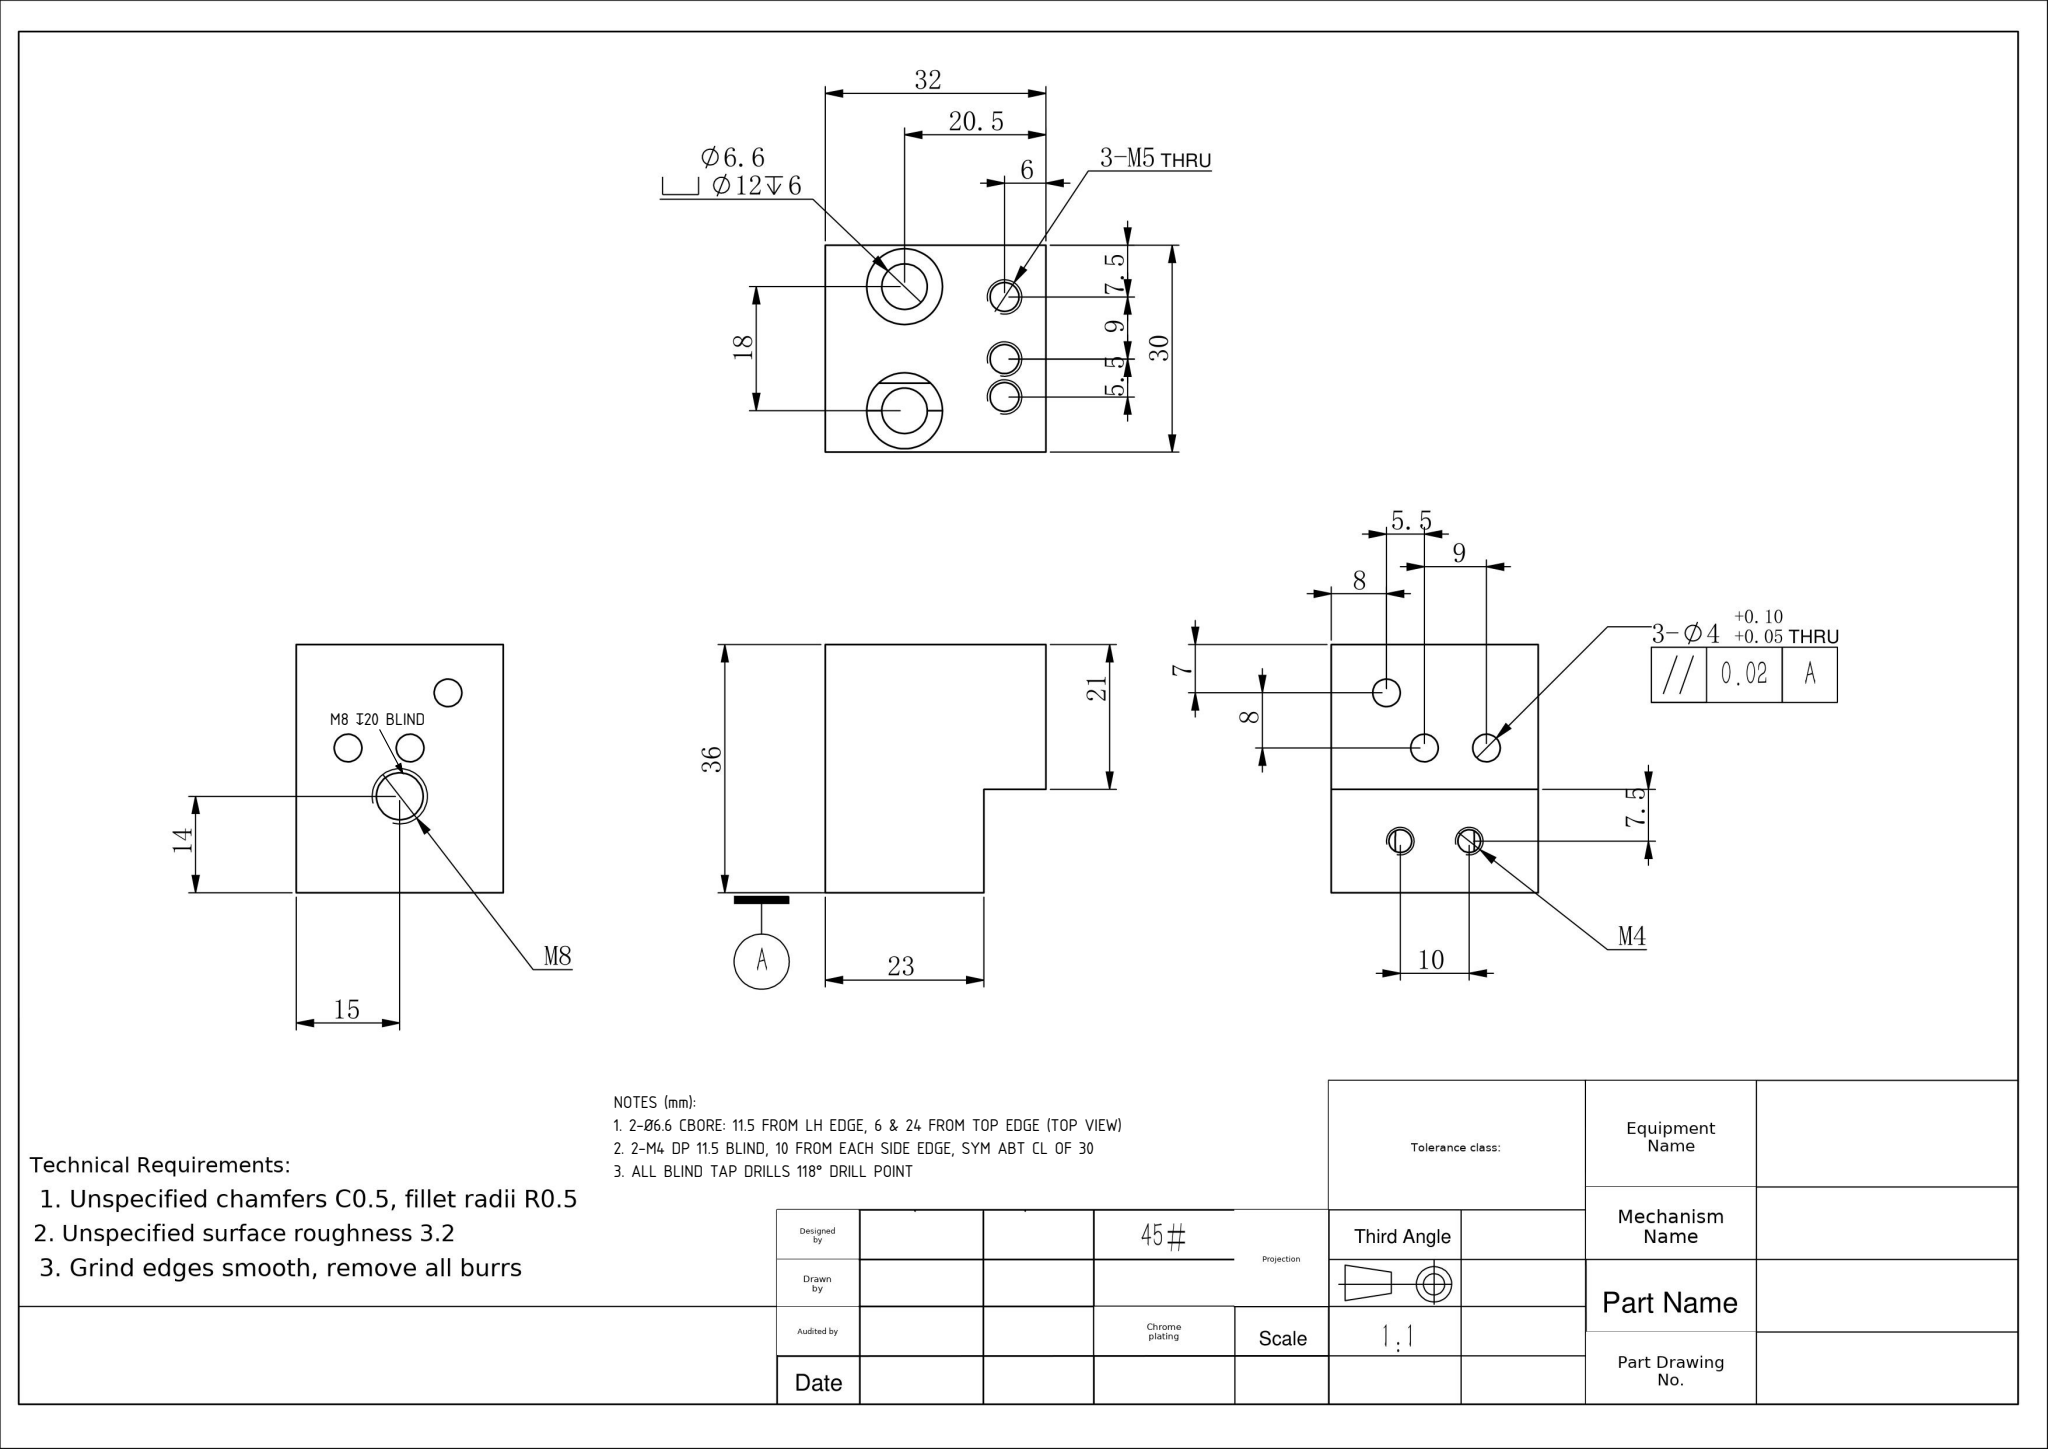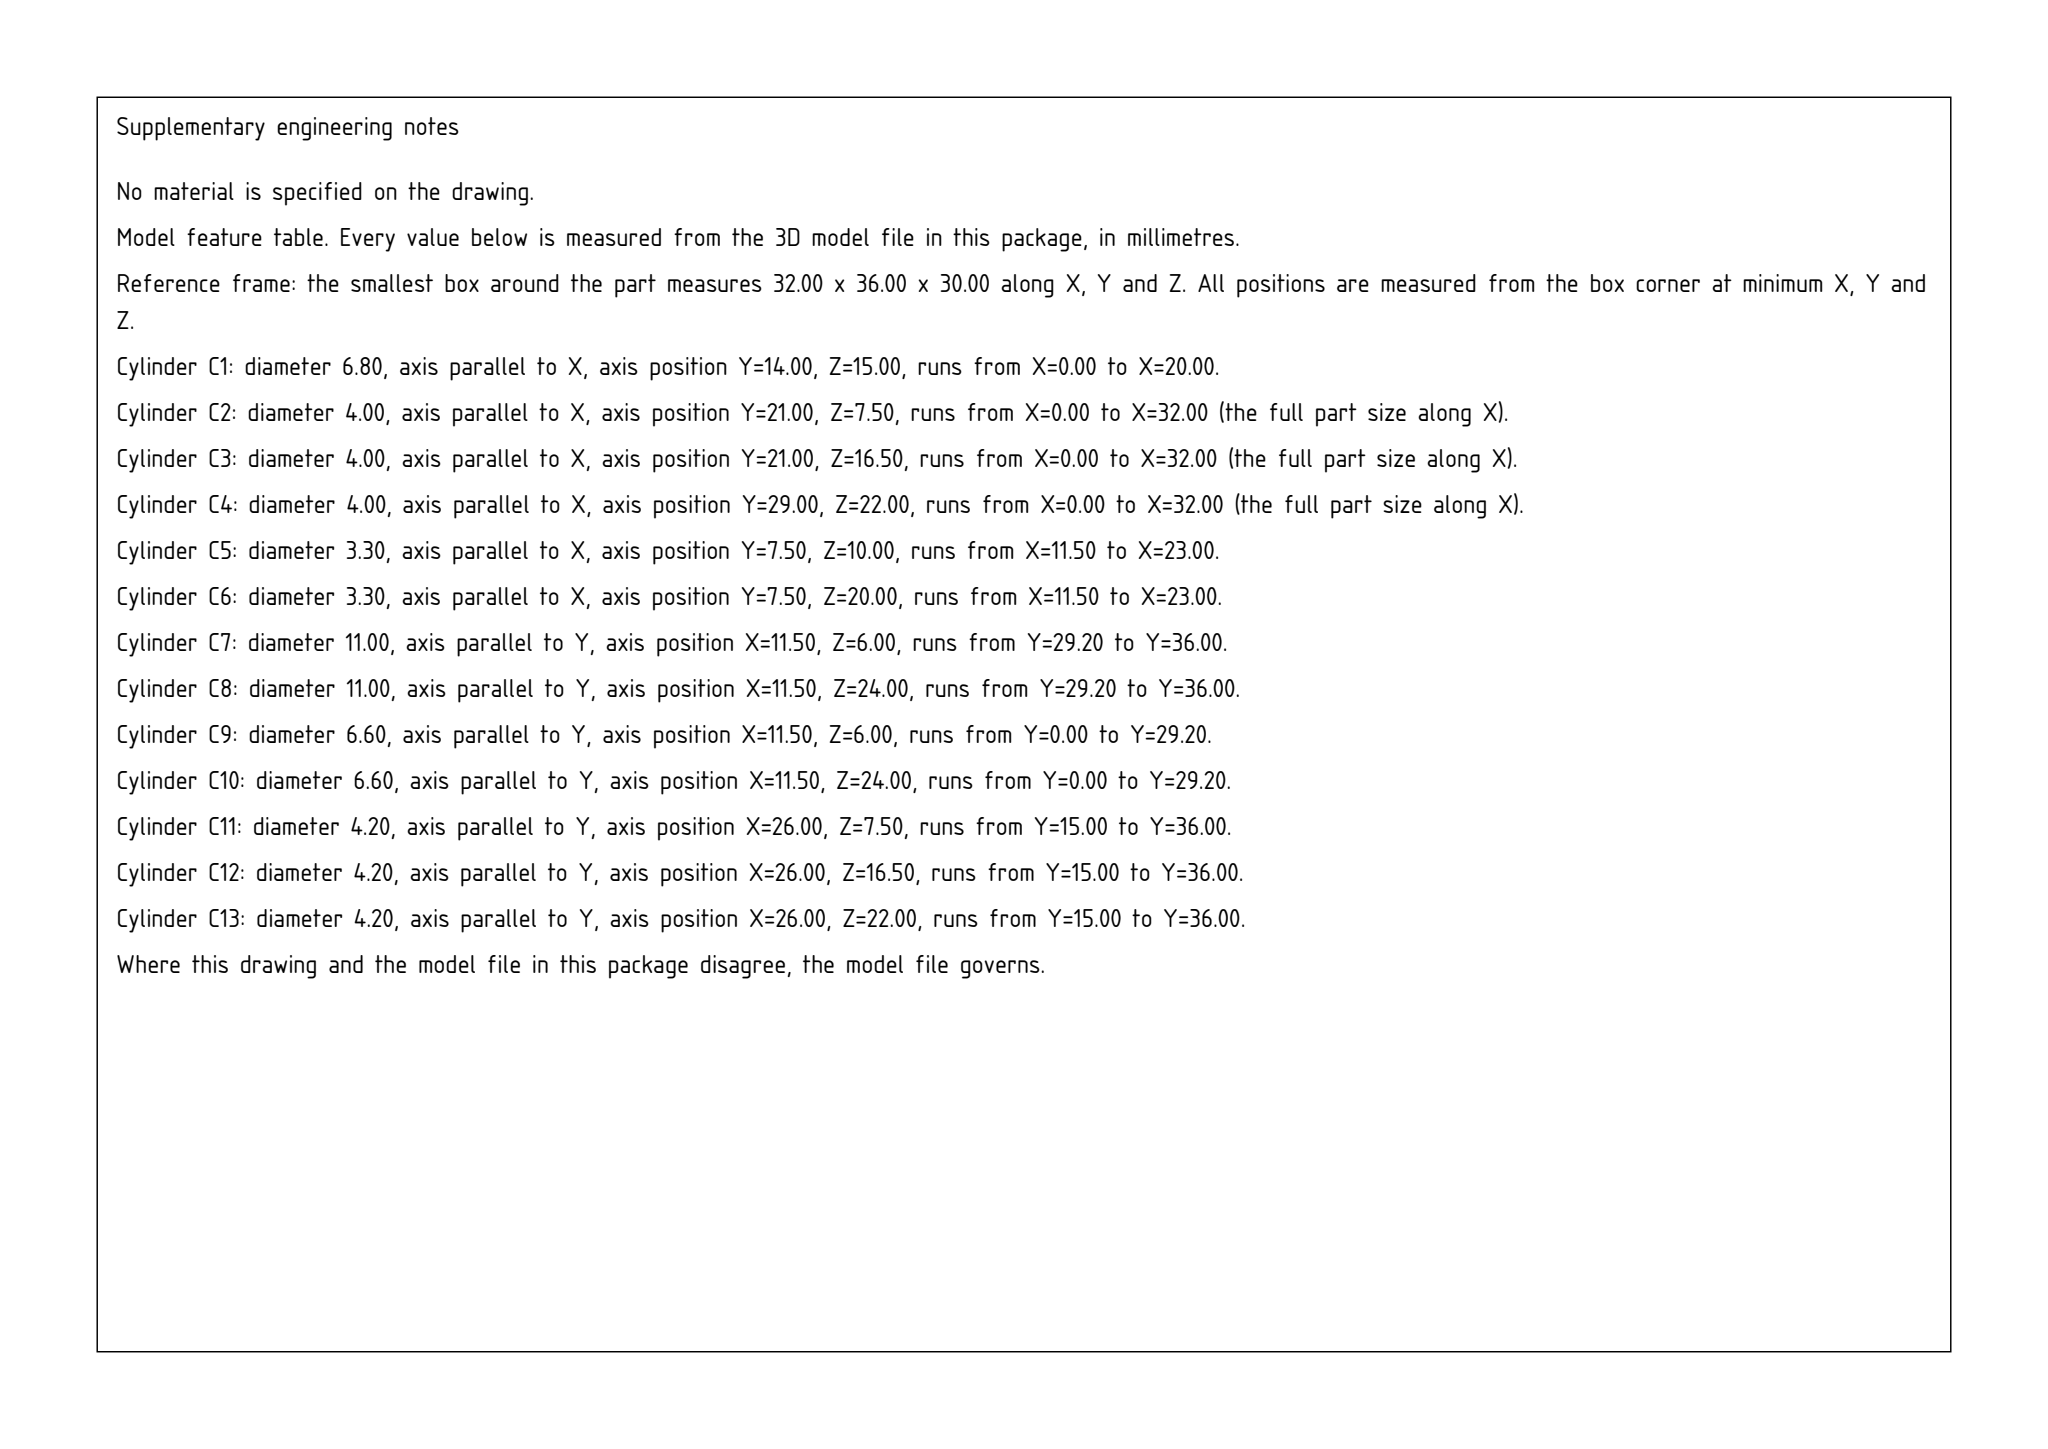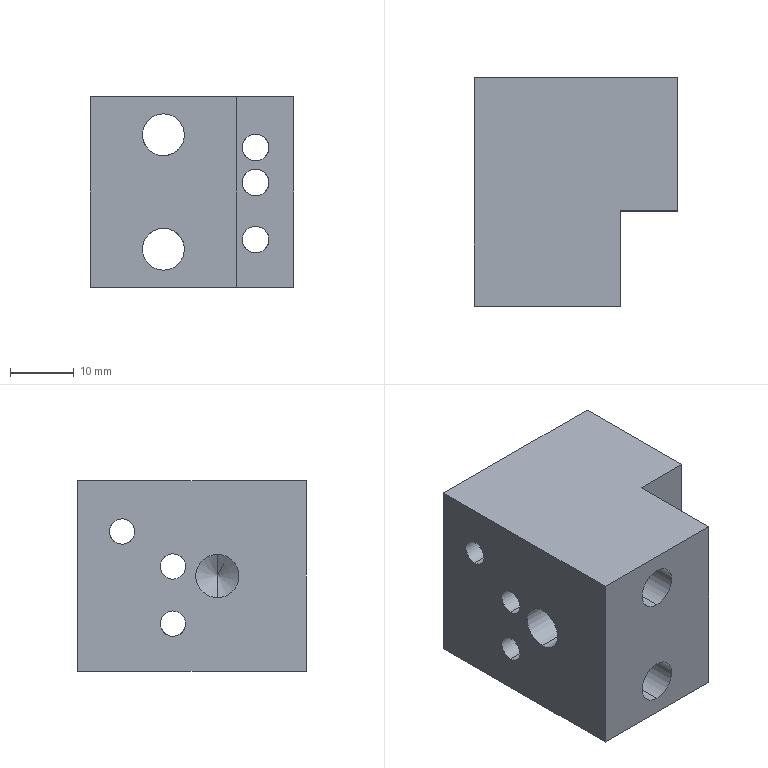Part | SolidWorks | mm | material 45# | 1 solid | 49 faces | box 32 x 36 x 30 mm | volume 24484 mm3 | cylinder 32 | plane 11 | cone 6 | commonest cylinder face diameters 4 x12 4.2 x6 3.3 x4 11 x4 6.6 x4 6.8 x2
Drawing notes:
2-Ø6.6 CBORE: 11.5 FROM LH EDGE, 6 & 24 FROM TOP EDGE (TOP VIEW) | from the solid: Ø6.6 y-axis cyls at x=11.5, z=6.0 and z=24.0 (18 apart) in 32x30 face
M8 DP 20 BLIND (LEFT VIEW) | from the solid: Ø6.8 x-axis tap drill at y=14, z=15, length 20 blind + 118° point
2-M4 DP 11.5 BLIND, 10 FROM EACH SIDE EDGE, SYM ABT CL OF 30 | from the solid: Ø3.3 x-axis tap drills at y=7.5, z=10.0 & z=20.0 of 30 width, length 11.5
ALL BLIND TAP DRILLS 118° DRILL POINT | from the solid: cones 118° on Ø3.3 (x4) and Ø6.8 (x2) drill ends